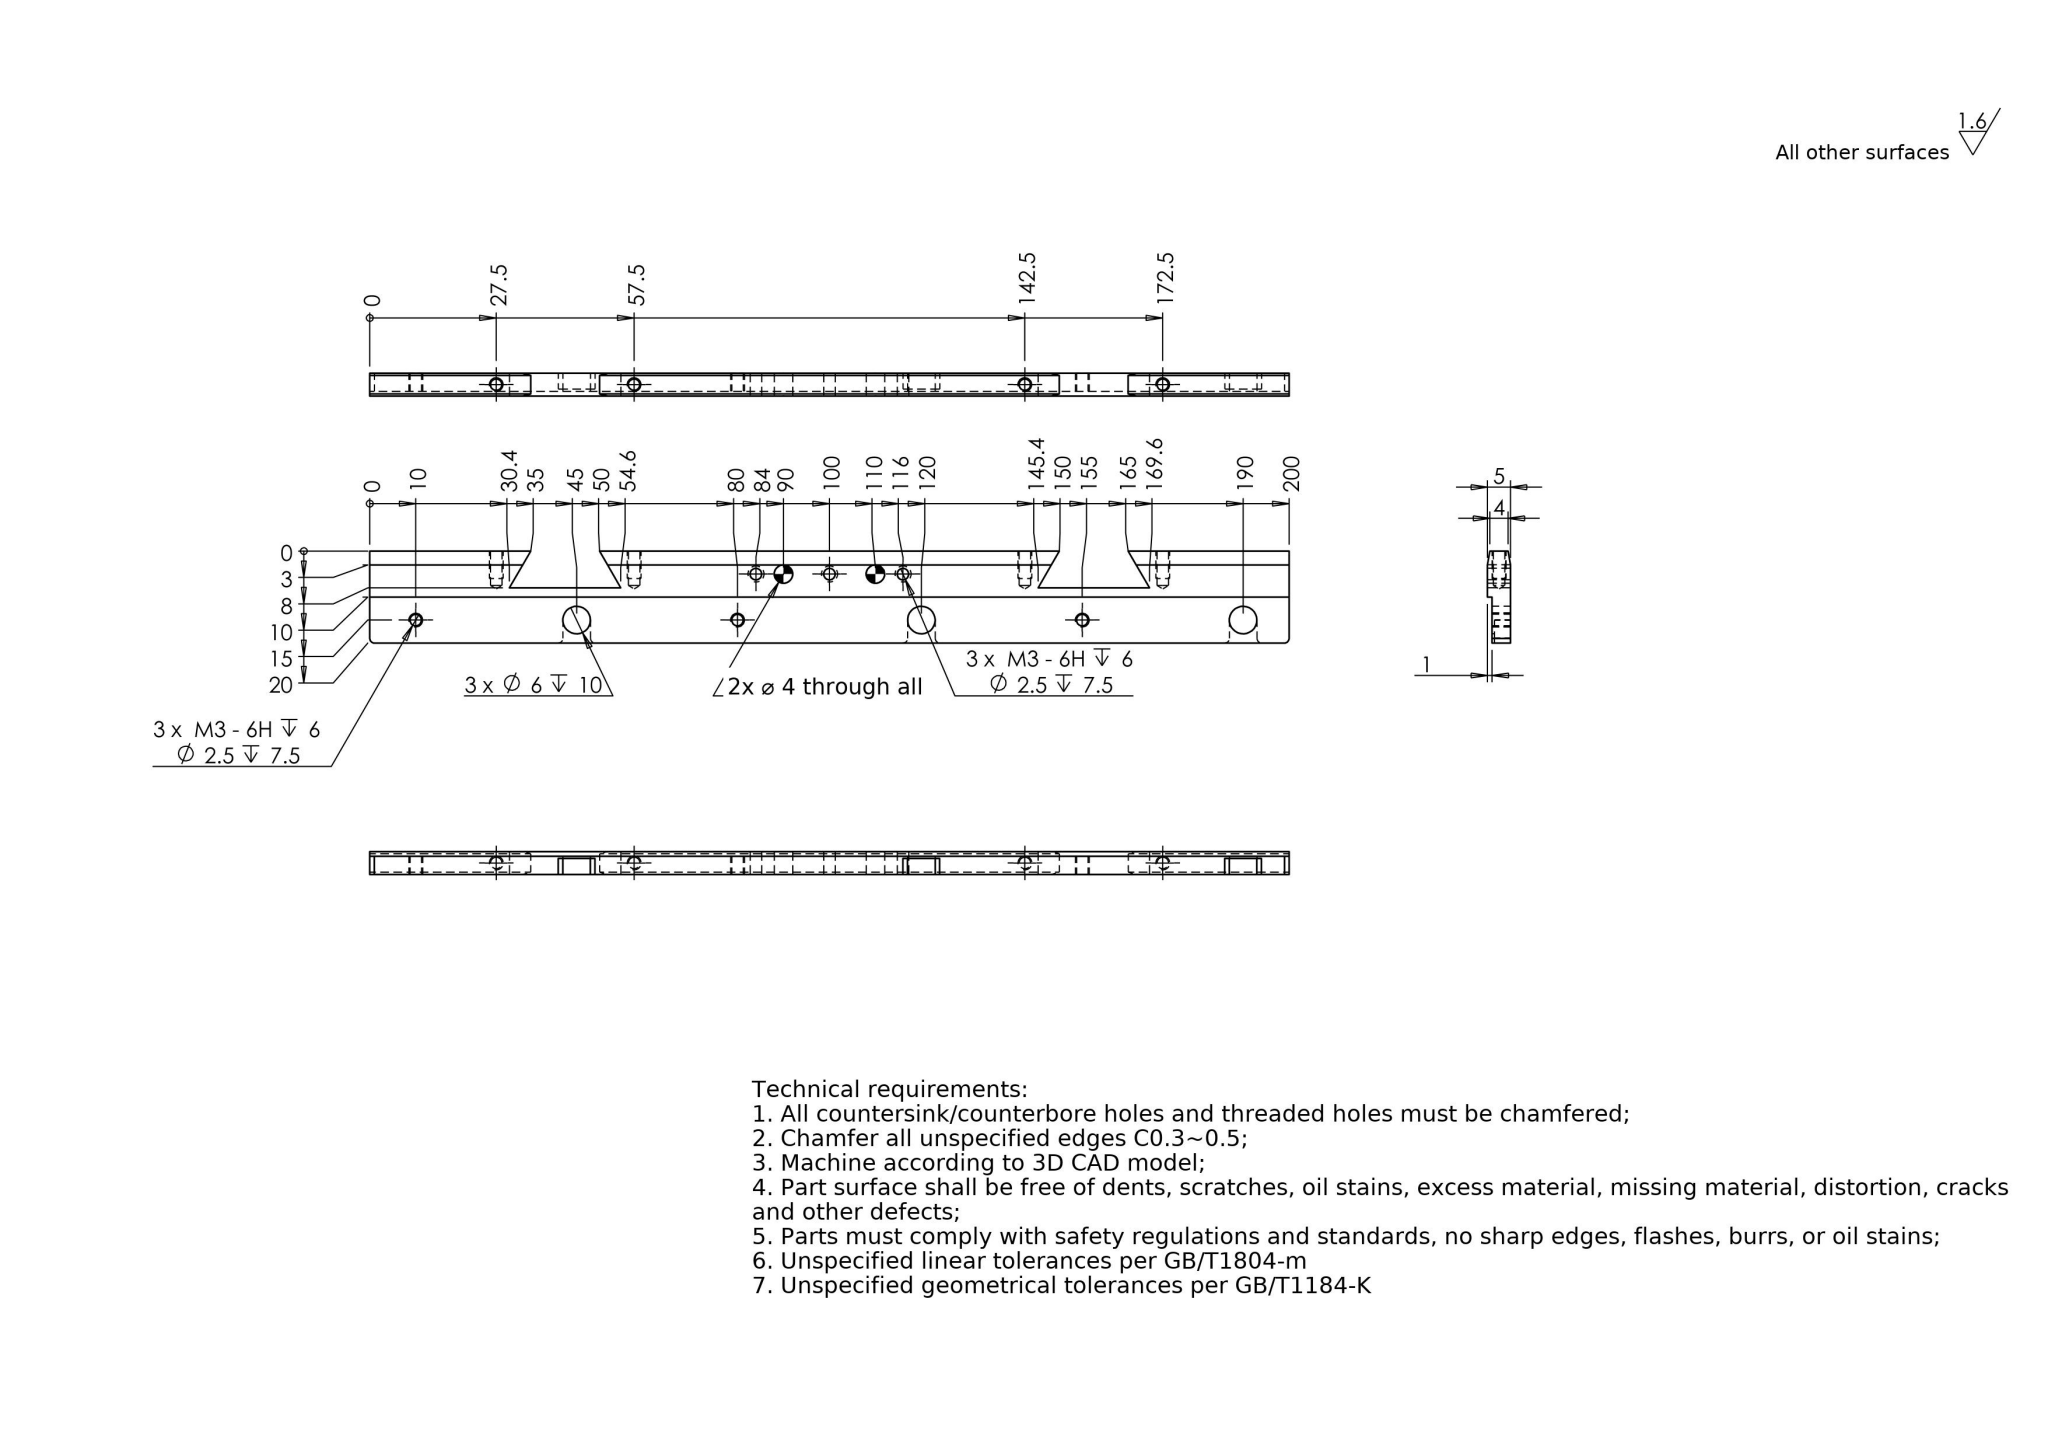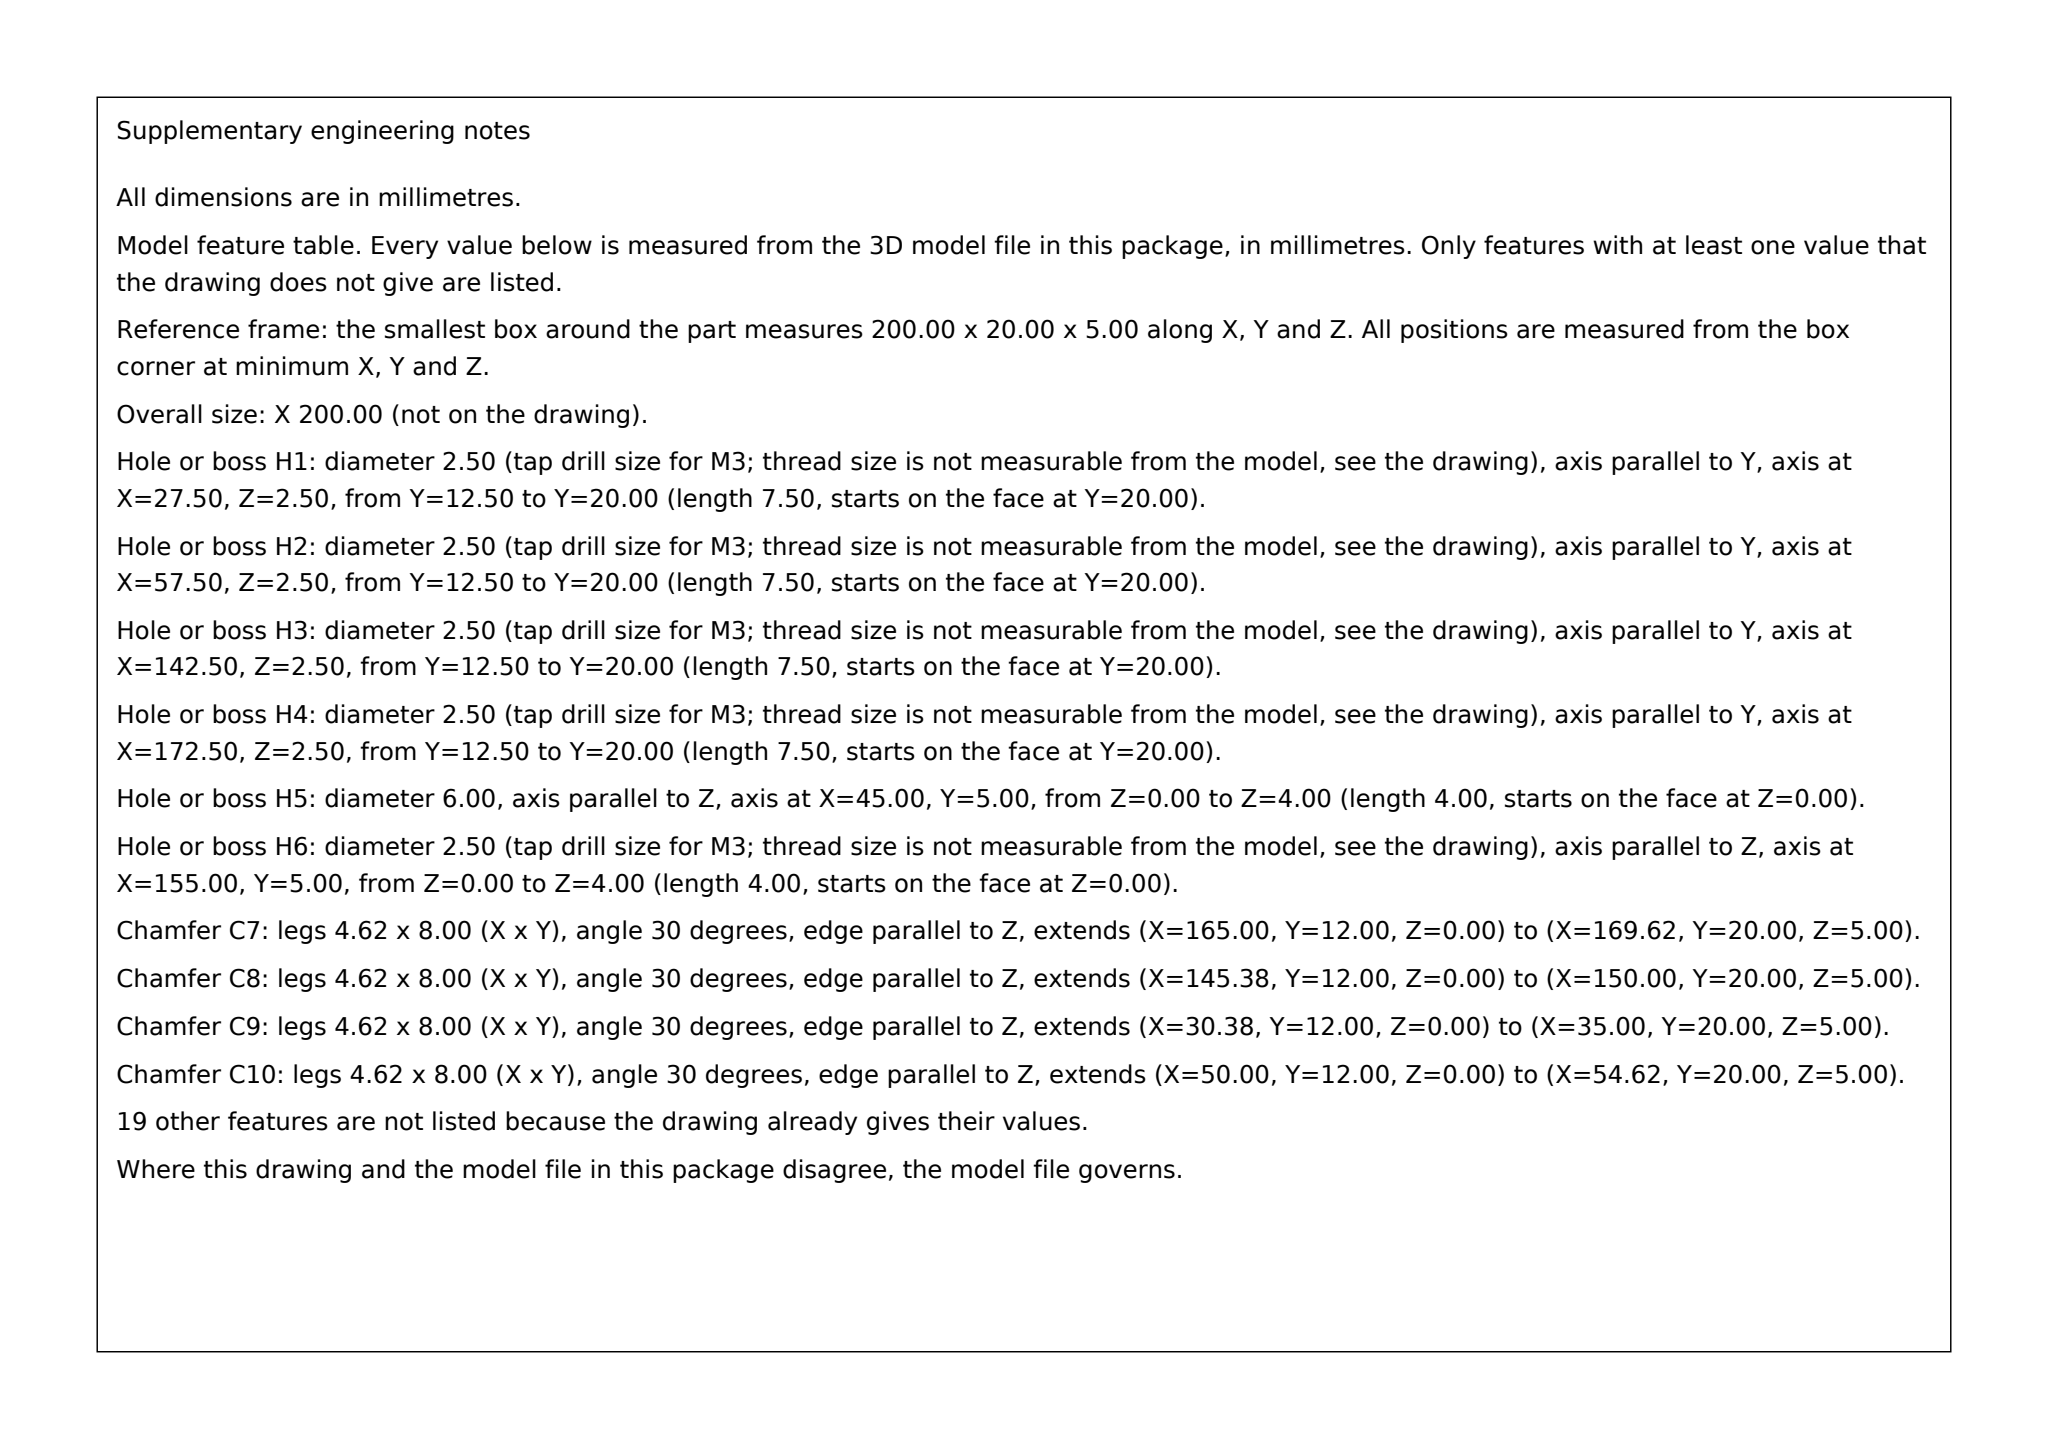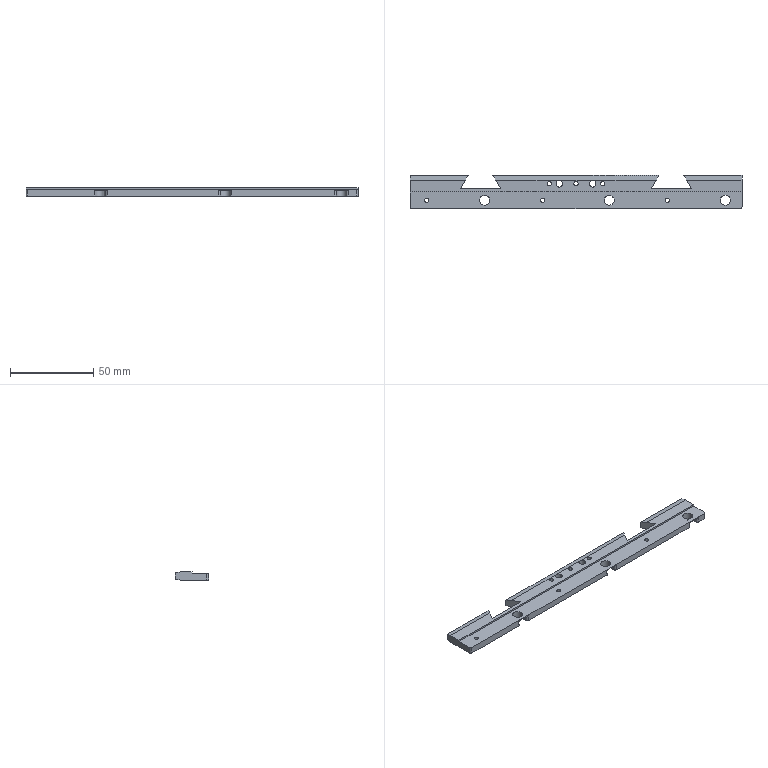Part | SolidWorks | mm | 1 solid | 77 faces | box 200 x 20 x 5 mm | volume 15255 mm3 | cylinder 38 | plane 31 | cone 8 | commonest cylinder face diameters 2.5 x20 2 x8 6 x6 4.02 x4
build123d program:
from build123d import *
from OCP.BRepFilletAPI import BRepFilletAPI_MakeChamfer

# Parameters (mm, degrees)
SKETCH1_W                    = 200
SKETCH1_H                    = 20
BOSS_EXTRUDE1_DEPTH          = 5
SKETCH2_W                    = 200
SKETCH2_H                    = 10
CUT_EXTRUDE1_DEPTH           = 1
M3_TAPPED_HOLE1_D            = 2.5
M3_TAPPED_HOLE1_DEPTH        = 7.5
M3_TAPPED_HOLE1_TIP          = 0.7511
F_6_0_6_DIAMETER_HOLE1_D     = 6
F_6_0_6_DIAMETER_HOLE1_DEPTH = 10
CUT_EXTRUDE2_DEPTH           = 3.5
FILLET1_R                    = 1
CUT_EXTRUDE3_DEPTH           = 101.623
M3_TAPPED_HOLE2_D            = 2.5
M3_TAPPED_HOLE2_DEPTH        = 7.5
M3_TAPPED_HOLE2_TIP          = 0.7511
CHAMFER1_SIZE                = 0.5
CHAMFER1_SIZE2               = 3
CHAMFER2_SIZE                = 3
CHAMFER2_SIZE2               = 0.5
F_4_0_4_DIAMETER_HOLE1_D     = 4.02
M3_TAPPED_HOLE3_D            = 2.5
M3_TAPPED_HOLE3_DEPTH        = 7.5
M3_TAPPED_HOLE3_TIP          = 0.7511


with BuildPart() as part:
    # Sketch1 → Boss-Extrude1 (new body)
    with BuildSketch(Plane.XY):
        Rectangle(SKETCH1_W, SKETCH1_H)
    extrude(amount=BOSS_EXTRUDE1_DEPTH)

    # Sketch2 → Cut-Extrude1 (cut)
    with BuildSketch(Plane.XY.offset(5)):
        with Locations((0, -5)):
            Rectangle(SKETCH2_W, SKETCH2_H)
    extrude(amount=-CUT_EXTRUDE1_DEPTH, mode=Mode.SUBTRACT)

    # M3 Tapped Hole1
    with Locations(Plane.XY.offset(4)):
        with Locations((-90, -5), (-20, -5), (55, -5)):
            Hole(M3_TAPPED_HOLE1_D / 2, depth=M3_TAPPED_HOLE1_DEPTH)
            with Locations((0, 0, -(M3_TAPPED_HOLE1_DEPTH + M3_TAPPED_HOLE1_TIP / 2))):  # 118° drill point
                Cone(0, M3_TAPPED_HOLE1_D / 2, M3_TAPPED_HOLE1_TIP, mode=Mode.SUBTRACT)

    # 6.0 _6_ Diameter Hole1
    with Locations(Plane.XY.offset(4)):
        with Locations((-55, -5), (20, -5), (90, -5)):
            Hole(F_6_0_6_DIAMETER_HOLE1_D / 2, depth=F_6_0_6_DIAMETER_HOLE1_DEPTH)

    # Sketch7 → Cut-Extrude2 (cut)
    with BuildSketch(Plane(origin=(0, 0, 0), x_dir=(-1, 0, 0), z_dir=(0, 0, -1))):
        with BuildLine():
            Line((-87, -5), (-87, -10))
            ThreePointArc((-87, -10), (-90, -13), (-93, -10))
            Line((-93, -10), (-93, -5))
            ThreePointArc((-93, -5), (-90, -2), (-87, -5))
        make_face()
        with BuildLine():
            Line((-17, -5), (-17, -10))
            ThreePointArc((-17, -10), (-20, -13), (-23, -10))
            Line((-23, -10), (-23, -5))
            ThreePointArc((-23, -5), (-20, -2), (-17, -5))
        make_face()
        with BuildLine():
            Line((58, -5), (58, -10))
            ThreePointArc((58, -10), (55, -13), (52, -10))
            Line((52, -10), (52, -5))
            ThreePointArc((52, -5), (55, -2), (58, -5))
        make_face()
    extrude(amount=-CUT_EXTRUDE2_DEPTH, mode=Mode.SUBTRACT)

    # Fillet1
    fillet1_edges = [part.edges().sort_by_distance(p)[0] for p in [
        (-58, -10, 1.75),
        (-52, -10, 1.75),
        (100, -10, 2),
        (-100, -10, 2),
        (87, -10, 1.75),
        (93, -10, 1.75),
        (17, -10, 1.75),
        (23, -10, 1.75),
    ]]
    fillet(fillet1_edges, radius=FILLET1_R)

    # Sketch8 → Cut-Extrude3 (cut, through all)
    with BuildSketch(Plane(origin=(0, 0, 0), x_dir=(-1, 0, 0), z_dir=(0, 0, -1))):
        Polygon((-69.619, 2), (-45.381, 2), (-50, 10), (-65, 10), align=None)
        Polygon((65, 10), (69.619, 2), (45.381, 2), (50, 10), align=None)
    extrude(amount=-CUT_EXTRUDE3_DEPTH, mode=Mode.SUBTRACT)

    # M3 Tapped Hole2
    with Locations(Plane(origin=(0, 10, 0), x_dir=(1, 0, 0), z_dir=(0, 1, 0))):
        with Locations((-72.5, -2.5), (72.5, -2.5), (42.5, -2.5), (-42.5, -2.5)):
            Hole(M3_TAPPED_HOLE2_D / 2, depth=M3_TAPPED_HOLE2_DEPTH)
            with Locations((0, 0, -(M3_TAPPED_HOLE2_DEPTH + M3_TAPPED_HOLE2_TIP / 2))):  # 118° drill point
                Cone(0, M3_TAPPED_HOLE2_D / 2, M3_TAPPED_HOLE2_TIP, mode=Mode.SUBTRACT)

    # Chamfer1: one chamfer whose edges measure the first distance from different faces: ONE call of the kernel's chamfer builder (chamfer() names one face for all edges)
    chamfer1_edges_1 = [part.edges().sort_by_distance(p)[0] for p in [
        (0, 10, 5),
    ]]
    chamfer1_side_1 = [part.faces().sort_by_distance(p)[0] for p in [
        (0, 10, 2.5),
    ]]
    chamfer1_edges_2 = [part.edges().sort_by_distance(p)[0] for p in [
        (-82.5, 10, 5),
    ]]
    chamfer1_side_2 = [part.faces().sort_by_distance(p)[0] for p in [
        (-82.789, 10, 2.5),
    ]]
    chamfer1_edges_3 = [part.edges().sort_by_distance(p)[0] for p in [
        (82.5, 10, 5),
    ]]
    chamfer1_side_3 = [part.faces().sort_by_distance(p)[0] for p in [
        (82.789, 10, 2.5),
    ]]
    chamfer1 = BRepFilletAPI_MakeChamfer(part.part.solid().wrapped)
    for e in chamfer1_edges_1:
        chamfer1.Add(CHAMFER1_SIZE, CHAMFER1_SIZE2, e.wrapped, chamfer1_side_1[0].wrapped)  # the first distance lies on this face
    for e in chamfer1_edges_2:
        chamfer1.Add(CHAMFER1_SIZE, CHAMFER1_SIZE2, e.wrapped, chamfer1_side_2[0].wrapped)  # the first distance lies on this face
    for e in chamfer1_edges_3:
        chamfer1.Add(CHAMFER1_SIZE, CHAMFER1_SIZE2, e.wrapped, chamfer1_side_3[0].wrapped)  # the first distance lies on this face
    add(Compound.cast(chamfer1.Shape()), mode=Mode.REPLACE)

    # Chamfer2
    chamfer2_edges = [part.edges().sort_by_distance(p)[0] for p in [
        (0, 10, 0),
        (-82.5, 10, 0),
        (82.5, 10, 0),
    ]]
    chamfer2_side = [part.faces().sort_by_distance(p)[0] for p in [
        (-0.6166, -0.2435, 0),
    ]]
    chamfer(chamfer2_edges, length=CHAMFER2_SIZE, length2=CHAMFER2_SIZE2, reference=chamfer2_side[0])

    # 4.0 _4_ Diameter Hole1 (through all)
    with Locations(Plane(origin=(0, 0, 0), x_dir=(-1, 0, 0), z_dir=(0, 0, -1))):
        with Locations((10, 5), (-10, 5)):
            Hole(F_4_0_4_DIAMETER_HOLE1_D / 2)

    # M3 Tapped Hole3
    with Locations(Plane(origin=(0, 0, 0), x_dir=(-1, 0, 0), z_dir=(0, 0, -1))):
        with Locations((16, 5), (0, 5), (-16, 5)):
            Hole(M3_TAPPED_HOLE3_D / 2, depth=M3_TAPPED_HOLE3_DEPTH)
            with Locations((0, 0, -(M3_TAPPED_HOLE3_DEPTH + M3_TAPPED_HOLE3_TIP / 2))):  # 118° drill point
                Cone(0, M3_TAPPED_HOLE3_D / 2, M3_TAPPED_HOLE3_TIP, mode=Mode.SUBTRACT)


solid = part.part